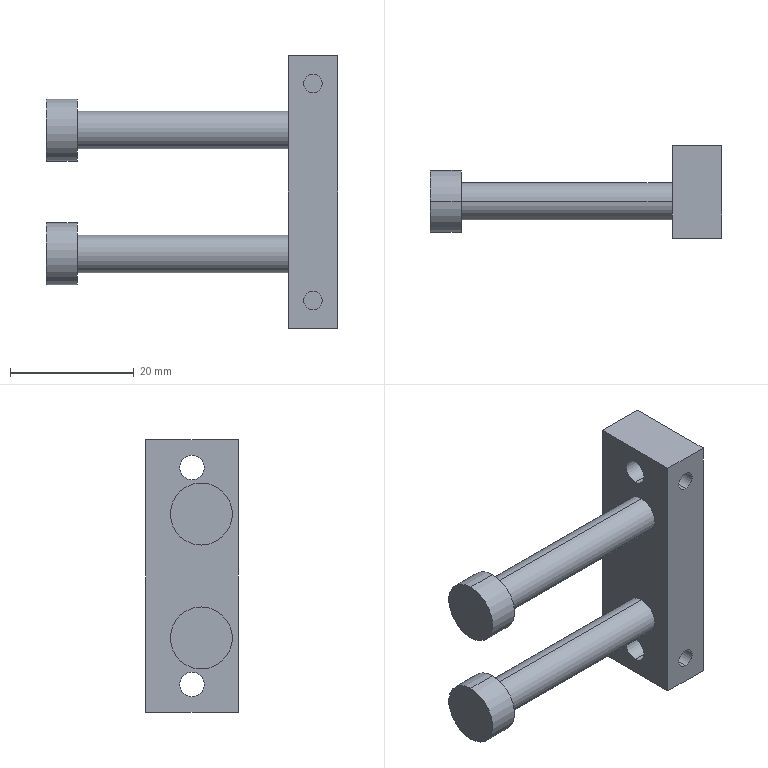Component | SolidWorks | F-YBExport-1-1_F-YBXCXSM10-15-Z73L-1_F-YBXCXSM10-15-Z73L_pr_cxs(PR_CXS_10-15)-1 | 1 solid | 34 faces | box 47 x 15 x 44 mm | volume 7646 mm3 | cylinder 20 | plane 14 | commonest cylinder face diameters 3 x8 10 x4 4 x4 6 x4
STEP:
#1=COLOUR_RGB('',0.7922,0.8196,0.9333);
#2=FILL_AREA_STYLE_COLOUR('',#1);
#3=FILL_AREA_STYLE('',(#2));
#4=SURFACE_STYLE_FILL_AREA(#3);
#5=SURFACE_SIDE_STYLE('',(#4));
#6=SURFACE_STYLE_USAGE(.BOTH.,#5);
#7=PRESENTATION_STYLE_ASSIGNMENT((#6));
#8=CARTESIAN_POINT('',(15.642,14.22,7.558));
#9=VERTEX_POINT('',#8);
#10=CARTESIAN_POINT('',(15.642,14.22,7.676));
#11=VERTEX_POINT('',#10);
#12=CARTESIAN_POINT('',(15.642,14.22,7.617));
#13=DIRECTION('',(0.,1.,0.));
#14=DIRECTION('',(0.,0.,-1.));
#15=AXIS2_PLACEMENT_3D('',#12,#13,#14);
#16=CIRCLE('',#15,0.05906);
#17=EDGE_CURVE('',#9,#11,#16,.T.);
#18=ORIENTED_EDGE('',*,*,#17,.T.);
#19=CARTESIAN_POINT('',(15.642,14.023,7.676));
#20=VERTEX_POINT('',#19);
#21=CARTESIAN_POINT('',(15.642,14.22,7.676));
#22=DIRECTION('',(0.,-1.,0.));
#23=VECTOR('',#22,39.37);
#24=LINE('',#21,#23);
#25=EDGE_CURVE('',#11,#20,#24,.T.);
#26=ORIENTED_EDGE('',*,*,#25,.T.);
#27=CARTESIAN_POINT('',(15.642,14.023,7.558));
#28=VERTEX_POINT('',#27);
#29=CARTESIAN_POINT('',(15.642,14.023,7.617));
#30=DIRECTION('',(0.,1.,0.));
#31=DIRECTION('',(0.,0.,-1.));
#32=AXIS2_PLACEMENT_3D('',#29,#30,#31);
#33=CIRCLE('',#32,0.05906);
#34=EDGE_CURVE('',#28,#20,#33,.T.);
#35=ORIENTED_EDGE('',*,*,#34,.F.);
#36=CARTESIAN_POINT('',(15.642,14.22,7.558));
#37=DIRECTION('',(0.,-1.,0.));
#38=VECTOR('',#37,39.37);
#39=LINE('',#36,#38);
#40=EDGE_CURVE('',#9,#28,#39,.T.);
#41=ORIENTED_EDGE('',*,*,#40,.F.);
#42=EDGE_LOOP('',(#18,#26,#35,#41));
#43=FACE_OUTER_BOUND('',#42,.T.);
#44=CARTESIAN_POINT('',(15.642,14.22,7.617));
#45=DIRECTION('',(0.,-1.,0.));
#46=DIRECTION('',(0.,0.,-1.));
#47=AXIS2_PLACEMENT_3D('',#44,#45,#46);
#48=CYLINDRICAL_SURFACE('',#47,0.05906);
#49=ADVANCED_FACE('',(#43),#48,.F.);
#50=CARTESIAN_POINT('',(15.642,14.22,6.18));
#51=VERTEX_POINT('',#50);
#52=CARTESIAN_POINT('',(15.642,14.22,6.298));
#53=VERTEX_POINT('',#52);
#54=CARTESIAN_POINT('',(15.642,14.22,6.239));
#55=DIRECTION('',(0.,1.,0.));
#56=DIRECTION('',(0.,0.,1.));
#57=AXIS2_PLACEMENT_3D('',#54,#55,#56);
#58=CIRCLE('',#57,0.05906);
#59=EDGE_CURVE('',#51,#53,#58,.T.);
#60=ORIENTED_EDGE('',*,*,#59,.T.);
#61=CARTESIAN_POINT('',(15.642,14.023,6.298));
#62=VERTEX_POINT('',#61);
#63=CARTESIAN_POINT('',(15.642,14.22,6.298));
#64=DIRECTION('',(0.,-1.,0.));
#65=VECTOR('',#64,39.37);
#66=LINE('',#63,#65);
#67=EDGE_CURVE('',#53,#62,#66,.T.);
#68=ORIENTED_EDGE('',*,*,#67,.T.);
#69=CARTESIAN_POINT('',(15.642,14.023,6.18));
#70=VERTEX_POINT('',#69);
#71=CARTESIAN_POINT('',(15.642,14.023,6.239));
#72=DIRECTION('',(0.,1.,0.));
#73=DIRECTION('',(0.,0.,1.));
#74=AXIS2_PLACEMENT_3D('',#71,#72,#73);
#75=CIRCLE('',#74,0.05906);
#76=EDGE_CURVE('',#70,#62,#75,.T.);
#77=ORIENTED_EDGE('',*,*,#76,.F.);
#78=CARTESIAN_POINT('',(15.642,14.22,6.18));
#79=DIRECTION('',(0.,-1.,0.));
#80=VECTOR('',#79,39.37);
#81=LINE('',#78,#80);
#82=EDGE_CURVE('',#51,#70,#81,.T.);
#83=ORIENTED_EDGE('',*,*,#82,.F.);
#84=EDGE_LOOP('',(#60,#68,#77,#83));
#85=FACE_OUTER_BOUND('',#84,.T.);
#86=CARTESIAN_POINT('',(15.642,14.22,6.239));
#87=DIRECTION('',(0.,-1.,0.));
#88=DIRECTION('',(0.,0.,-1.));
#89=AXIS2_PLACEMENT_3D('',#86,#87,#88);
#90=CYLINDRICAL_SURFACE('',#89,0.05906);
#91=ADVANCED_FACE('',(#85),#90,.F.);
#92=CARTESIAN_POINT('',(15.642,14.416,7.558));
#93=VERTEX_POINT('',#92);
#94=CARTESIAN_POINT('',(15.642,14.416,7.676));
#95=VERTEX_POINT('',#94);
#96=CARTESIAN_POINT('',(15.642,14.416,7.617));
#97=DIRECTION('',(0.,1.,0.));
#98=DIRECTION('',(0.,0.,-1.));
#99=AXIS2_PLACEMENT_3D('',#96,#97,#98);
#100=CIRCLE('',#99,0.05906);
#101=EDGE_CURVE('',#93,#95,#100,.T.);
#102=ORIENTED_EDGE('',*,*,#101,.F.);
#103=CARTESIAN_POINT('',(15.642,14.613,7.558));
#104=VERTEX_POINT('',#103);
#105=CARTESIAN_POINT('',(15.642,14.416,7.558));
#106=DIRECTION('',(0.,1.,0.));
#107=VECTOR('',#106,39.37);
#108=LINE('',#105,#107);
#109=EDGE_CURVE('',#93,#104,#108,.T.);
#110=ORIENTED_EDGE('',*,*,#109,.T.);
#111=CARTESIAN_POINT('',(15.642,14.613,7.676));
#112=VERTEX_POINT('',#111);
#113=CARTESIAN_POINT('',(15.642,14.613,7.617));
#114=DIRECTION('',(0.,1.,0.));
#115=DIRECTION('',(0.,0.,-1.));
#116=AXIS2_PLACEMENT_3D('',#113,#114,#115);
#117=CIRCLE('',#116,0.05906);
#118=EDGE_CURVE('',#104,#112,#117,.T.);
#119=ORIENTED_EDGE('',*,*,#118,.T.);
#120=CARTESIAN_POINT('',(15.642,14.416,7.676));
#121=DIRECTION('',(0.,1.,0.));
#122=VECTOR('',#121,39.37);
#123=LINE('',#120,#122);
#124=EDGE_CURVE('',#95,#112,#123,.T.);
#125=ORIENTED_EDGE('',*,*,#124,.F.);
#126=EDGE_LOOP('',(#102,#110,#119,#125));
#127=FACE_OUTER_BOUND('',#126,.T.);
#128=CARTESIAN_POINT('',(15.642,14.416,7.617));
#129=DIRECTION('',(0.,1.,0.));
#130=DIRECTION('',(0.,0.,1.));
#131=AXIS2_PLACEMENT_3D('',#128,#129,#130);
#132=CYLINDRICAL_SURFACE('',#131,0.05906);
#133=ADVANCED_FACE('',(#127),#132,.F.);
#134=CARTESIAN_POINT('',(15.642,14.416,6.18));
#135=VERTEX_POINT('',#134);
#136=CARTESIAN_POINT('',(15.642,14.416,6.298));
#137=VERTEX_POINT('',#136);
#138=CARTESIAN_POINT('',(15.642,14.416,6.239));
#139=DIRECTION('',(0.,1.,0.));
#140=DIRECTION('',(0.,0.,1.));
#141=AXIS2_PLACEMENT_3D('',#138,#139,#140);
#142=CIRCLE('',#141,0.05906);
#143=EDGE_CURVE('',#135,#137,#142,.T.);
#144=ORIENTED_EDGE('',*,*,#143,.F.);
#145=CARTESIAN_POINT('',(15.642,14.613,6.18));
#146=VERTEX_POINT('',#145);
#147=CARTESIAN_POINT('',(15.642,14.416,6.18));
#148=DIRECTION('',(0.,1.,0.));
#149=VECTOR('',#148,39.37);
#150=LINE('',#147,#149);
#151=EDGE_CURVE('',#135,#146,#150,.T.);
#152=ORIENTED_EDGE('',*,*,#151,.T.);
#153=CARTESIAN_POINT('',(15.642,14.613,6.298));
#154=VERTEX_POINT('',#153);
#155=CARTESIAN_POINT('',(15.642,14.613,6.239));
#156=DIRECTION('',(0.,1.,0.));
#157=DIRECTION('',(0.,0.,1.));
#158=AXIS2_PLACEMENT_3D('',#155,#156,#157);
#159=CIRCLE('',#158,0.05906);
#160=EDGE_CURVE('',#146,#154,#159,.T.);
#161=ORIENTED_EDGE('',*,*,#160,.T.);
#162=CARTESIAN_POINT('',(15.642,14.416,6.298));
#163=DIRECTION('',(0.,1.,0.));
#164=VECTOR('',#163,39.37);
#165=LINE('',#162,#164);
#166=EDGE_CURVE('',#137,#154,#165,.T.);
#167=ORIENTED_EDGE('',*,*,#166,.F.);
#168=EDGE_LOOP('',(#144,#152,#161,#167));
#169=FACE_OUTER_BOUND('',#168,.T.);
#170=CARTESIAN_POINT('',(15.642,14.416,6.239));
#171=DIRECTION('',(0.,1.,0.));
#172=DIRECTION('',(0.,0.,1.));
#173=AXIS2_PLACEMENT_3D('',#170,#171,#172);
#174=CYLINDRICAL_SURFACE('',#173,0.05906);
#175=ADVANCED_FACE('',(#169),#174,.F.);
#176=CARTESIAN_POINT('',(14.146,14.259,7.519));
#177=VERTEX_POINT('',#176);
#178=CARTESIAN_POINT('',(14.146,14.259,7.125));
#179=VERTEX_POINT('',#178);
#180=CARTESIAN_POINT('',(14.146,14.259,7.322));
#181=DIRECTION('',(-1.,0.,0.));
#182=DIRECTION('',(0.,0.,1.));
#183=AXIS2_PLACEMENT_3D('',#180,#181,#182);
#184=CIRCLE('',#183,0.1969);
#185=EDGE_CURVE('',#177,#179,#184,.T.);
#186=ORIENTED_EDGE('',*,*,#185,.T.);
#187=CARTESIAN_POINT('',(13.949,14.259,7.125));
#188=VERTEX_POINT('',#187);
#189=CARTESIAN_POINT('',(14.146,14.259,7.125));
#190=DIRECTION('',(-1.,0.,0.));
#191=VECTOR('',#190,39.37);
#192=LINE('',#189,#191);
#193=EDGE_CURVE('',#179,#188,#192,.T.);
#194=ORIENTED_EDGE('',*,*,#193,.T.);
#195=CARTESIAN_POINT('',(13.949,14.259,7.519));
#196=VERTEX_POINT('',#195);
#197=CARTESIAN_POINT('',(13.949,14.259,7.322));
#198=DIRECTION('',(-1.,0.,0.));
#199=DIRECTION('',(0.,0.,1.));
#200=AXIS2_PLACEMENT_3D('',#197,#198,#199);
#201=CIRCLE('',#200,0.1969);
#202=EDGE_CURVE('',#196,#188,#201,.T.);
#203=ORIENTED_EDGE('',*,*,#202,.F.);
#204=CARTESIAN_POINT('',(14.146,14.259,7.519));
#205=DIRECTION('',(-1.,0.,0.));
#206=VECTOR('',#205,39.37);
#207=LINE('',#204,#206);
#208=EDGE_CURVE('',#177,#196,#207,.T.);
#209=ORIENTED_EDGE('',*,*,#208,.F.);
#210=EDGE_LOOP('',(#186,#194,#203,#209));
#211=FACE_OUTER_BOUND('',#210,.T.);
#212=CARTESIAN_POINT('',(14.146,14.259,7.322));
#213=DIRECTION('',(-1.,0.,0.));
#214=DIRECTION('',(0.,0.,1.));
#215=AXIS2_PLACEMENT_3D('',#212,#213,#214);
#216=CYLINDRICAL_SURFACE('',#215,0.1969);
#217=ADVANCED_FACE('',(#211),#216,.T.);
#218=CARTESIAN_POINT('',(14.146,14.259,6.731));
#219=VERTEX_POINT('',#218);
#220=CARTESIAN_POINT('',(14.146,14.259,6.338));
#221=VERTEX_POINT('',#220);
#222=CARTESIAN_POINT('',(14.146,14.259,6.535));
#223=DIRECTION('',(-1.,0.,0.));
#224=DIRECTION('',(0.,0.,1.));
#225=AXIS2_PLACEMENT_3D('',#222,#223,#224);
#226=CIRCLE('',#225,0.1969);
#227=EDGE_CURVE('',#219,#221,#226,.T.);
#228=ORIENTED_EDGE('',*,*,#227,.T.);
#229=CARTESIAN_POINT('',(13.949,14.259,6.338));
#230=VERTEX_POINT('',#229);
#231=CARTESIAN_POINT('',(14.146,14.259,6.338));
#232=DIRECTION('',(-1.,0.,0.));
#233=VECTOR('',#232,39.37);
#234=LINE('',#231,#233);
#235=EDGE_CURVE('',#221,#230,#234,.T.);
#236=ORIENTED_EDGE('',*,*,#235,.T.);
#237=CARTESIAN_POINT('',(13.949,14.259,6.731));
#238=VERTEX_POINT('',#237);
#239=CARTESIAN_POINT('',(13.949,14.259,6.535));
#240=DIRECTION('',(-1.,0.,0.));
#241=DIRECTION('',(0.,0.,1.));
#242=AXIS2_PLACEMENT_3D('',#239,#240,#241);
#243=CIRCLE('',#242,0.1969);
#244=EDGE_CURVE('',#238,#230,#243,.T.);
#245=ORIENTED_EDGE('',*,*,#244,.F.);
#246=CARTESIAN_POINT('',(14.146,14.259,6.731));
#247=DIRECTION('',(-1.,0.,0.));
#248=VECTOR('',#247,39.37);
#249=LINE('',#246,#248);
#250=EDGE_CURVE('',#219,#238,#249,.T.);
#251=ORIENTED_EDGE('',*,*,#250,.F.);
#252=EDGE_LOOP('',(#228,#236,#245,#251));
#253=FACE_OUTER_BOUND('',#252,.T.);
#254=CARTESIAN_POINT('',(14.146,14.259,6.535));
#255=DIRECTION('',(-1.,0.,0.));
#256=DIRECTION('',(0.,0.,1.));
#257=AXIS2_PLACEMENT_3D('',#254,#255,#256);
#258=CYLINDRICAL_SURFACE('',#257,0.1969);
#259=ADVANCED_FACE('',(#253),#258,.T.);
#260=CARTESIAN_POINT('',(15.799,14.318,7.696));
#261=VERTEX_POINT('',#260);
#262=CARTESIAN_POINT('',(15.799,14.318,7.539));
#263=VERTEX_POINT('',#262);
#264=CARTESIAN_POINT('',(15.799,14.318,7.617));
#265=DIRECTION('',(1.,0.,0.));
#266=DIRECTION('',(0.,0.,-1.));
#267=AXIS2_PLACEMENT_3D('',#264,#265,#266);
#268=CIRCLE('',#267,0.07874);
#269=EDGE_CURVE('',#261,#263,#268,.T.);
#270=ORIENTED_EDGE('',*,*,#269,.T.);
#271=CARTESIAN_POINT('',(15.484,14.318,7.539));
#272=VERTEX_POINT('',#271);
#273=CARTESIAN_POINT('',(15.799,14.318,7.539));
#274=DIRECTION('',(-1.,0.,0.));
#275=VECTOR('',#274,39.37);
#276=LINE('',#273,#275);
#277=EDGE_CURVE('',#263,#272,#276,.T.);
#278=ORIENTED_EDGE('',*,*,#277,.T.);
#279=CARTESIAN_POINT('',(15.484,14.318,7.696));
#280=VERTEX_POINT('',#279);
#281=CARTESIAN_POINT('',(15.484,14.318,7.617));
#282=DIRECTION('',(1.,0.,0.));
#283=DIRECTION('',(0.,0.,-1.));
#284=AXIS2_PLACEMENT_3D('',#281,#282,#283);
#285=CIRCLE('',#284,0.07874);
#286=EDGE_CURVE('',#280,#272,#285,.T.);
#287=ORIENTED_EDGE('',*,*,#286,.F.);
#288=CARTESIAN_POINT('',(15.799,14.318,7.696));
#289=DIRECTION('',(-1.,0.,0.));
#290=VECTOR('',#289,39.37);
#291=LINE('',#288,#290);
#292=EDGE_CURVE('',#261,#280,#291,.T.);
#293=ORIENTED_EDGE('',*,*,#292,.F.);
#294=EDGE_LOOP('',(#270,#278,#287,#293));
#295=FACE_OUTER_BOUND('',#294,.T.);
#296=CARTESIAN_POINT('',(15.799,14.318,7.617));
#297=DIRECTION('',(-1.,0.,0.));
#298=DIRECTION('',(0.,0.,1.));
#299=AXIS2_PLACEMENT_3D('',#296,#297,#298);
#300=CYLINDRICAL_SURFACE('',#299,0.07874);
#301=ADVANCED_FACE('',(#295),#300,.F.);
#302=CARTESIAN_POINT('',(15.799,14.318,6.318));
#303=VERTEX_POINT('',#302);
#304=CARTESIAN_POINT('',(15.799,14.318,6.161));
#305=VERTEX_POINT('',#304);
#306=CARTESIAN_POINT('',(15.799,14.318,6.239));
#307=DIRECTION('',(1.,0.,0.));
#308=DIRECTION('',(0.,0.,-1.));
#309=AXIS2_PLACEMENT_3D('',#306,#307,#308);
#310=CIRCLE('',#309,0.07874);
#311=EDGE_CURVE('',#303,#305,#310,.T.);
#312=ORIENTED_EDGE('',*,*,#311,.T.);
#313=CARTESIAN_POINT('',(15.484,14.318,6.161));
#314=VERTEX_POINT('',#313);
#315=CARTESIAN_POINT('',(15.799,14.318,6.161));
#316=DIRECTION('',(-1.,0.,0.));
#317=VECTOR('',#316,39.37);
#318=LINE('',#315,#317);
#319=EDGE_CURVE('',#305,#314,#318,.T.);
#320=ORIENTED_EDGE('',*,*,#319,.T.);
#321=CARTESIAN_POINT('',(15.484,14.318,6.318));
#322=VERTEX_POINT('',#321);
#323=CARTESIAN_POINT('',(15.484,14.318,6.239));
#324=DIRECTION('',(1.,0.,0.));
#325=DIRECTION('',(0.,0.,-1.));
#326=AXIS2_PLACEMENT_3D('',#323,#324,#325);
#327=CIRCLE('',#326,0.07874);
#328=EDGE_CURVE('',#322,#314,#327,.T.);
#329=ORIENTED_EDGE('',*,*,#328,.F.);
#330=CARTESIAN_POINT('',(15.799,14.318,6.318));
#331=DIRECTION('',(-1.,0.,0.));
#332=VECTOR('',#331,39.37);
#333=LINE('',#330,#332);
#334=EDGE_CURVE('',#303,#322,#333,.T.);
#335=ORIENTED_EDGE('',*,*,#334,.F.);
#336=EDGE_LOOP('',(#312,#320,#329,#335));
#337=FACE_OUTER_BOUND('',#336,.T.);
#338=CARTESIAN_POINT('',(15.799,14.318,6.239));
#339=DIRECTION('',(-1.,0.,0.));
#340=DIRECTION('',(0.,0.,1.));
#341=AXIS2_PLACEMENT_3D('',#338,#339,#340);
#342=CYLINDRICAL_SURFACE('',#341,0.07874);
#343=ADVANCED_FACE('',(#337),#342,.F.);
#344=CARTESIAN_POINT('',(14.146,14.259,6.653));
#345=VERTEX_POINT('',#344);
#346=CARTESIAN_POINT('',(14.146,14.259,6.417));
#347=VERTEX_POINT('',#346);
#348=CARTESIAN_POINT('',(14.146,14.259,6.535));
#349=DIRECTION('',(-1.,0.,0.));
#350=DIRECTION('',(0.,0.,1.));
#351=AXIS2_PLACEMENT_3D('',#348,#349,#350);
#352=CIRCLE('',#351,0.1181);
#353=EDGE_CURVE('',#345,#347,#352,.T.);
#354=ORIENTED_EDGE('',*,*,#353,.F.);
#355=CARTESIAN_POINT('',(15.484,14.259,6.653));
#356=VERTEX_POINT('',#355);
#357=CARTESIAN_POINT('',(13.949,14.259,6.653));
#358=DIRECTION('',(1.,0.,0.));
#359=VECTOR('',#358,39.37);
#360=LINE('',#357,#359);
#361=EDGE_CURVE('',#345,#356,#360,.T.);
#362=ORIENTED_EDGE('',*,*,#361,.T.);
#363=CARTESIAN_POINT('',(15.484,14.259,6.417));
#364=VERTEX_POINT('',#363);
#365=CARTESIAN_POINT('',(15.484,14.259,6.535));
#366=DIRECTION('',(1.,0.,0.));
#367=DIRECTION('',(0.,0.,1.));
#368=AXIS2_PLACEMENT_3D('',#365,#366,#367);
#369=CIRCLE('',#368,0.1181);
#370=EDGE_CURVE('',#364,#356,#369,.T.);
#371=ORIENTED_EDGE('',*,*,#370,.F.);
#372=CARTESIAN_POINT('',(13.949,14.259,6.417));
#373=DIRECTION('',(1.,0.,0.));
#374=VECTOR('',#373,39.37);
#375=LINE('',#372,#374);
#376=EDGE_CURVE('',#347,#364,#375,.T.);
#377=ORIENTED_EDGE('',*,*,#376,.F.);
#378=EDGE_LOOP('',(#354,#362,#371,#377));
#379=FACE_OUTER_BOUND('',#378,.T.);
#380=CARTESIAN_POINT('',(13.949,14.259,6.535));
#381=DIRECTION('',(1.,0.,0.));
#382=DIRECTION('',(0.,0.,-1.));
#383=AXIS2_PLACEMENT_3D('',#380,#381,#382);
#384=CYLINDRICAL_SURFACE('',#383,0.1181);
#385=ADVANCED_FACE('',(#379),#384,.T.);
#386=CARTESIAN_POINT('',(14.146,14.259,7.44));
#387=VERTEX_POINT('',#386);
#388=CARTESIAN_POINT('',(14.146,14.259,7.204));
#389=VERTEX_POINT('',#388);
#390=CARTESIAN_POINT('',(14.146,14.259,7.322));
#391=DIRECTION('',(-1.,0.,0.));
#392=DIRECTION('',(0.,0.,1.));
#393=AXIS2_PLACEMENT_3D('',#390,#391,#392);
#394=CIRCLE('',#393,0.1181);
#395=EDGE_CURVE('',#387,#389,#394,.T.);
#396=ORIENTED_EDGE('',*,*,#395,.F.);
#397=CARTESIAN_POINT('',(15.484,14.259,7.44));
#398=VERTEX_POINT('',#397);
#399=CARTESIAN_POINT('',(13.949,14.259,7.44));
#400=DIRECTION('',(1.,0.,0.));
#401=VECTOR('',#400,39.37);
#402=LINE('',#399,#401);
#403=EDGE_CURVE('',#387,#398,#402,.T.);
#404=ORIENTED_EDGE('',*,*,#403,.T.);
#405=CARTESIAN_POINT('',(15.484,14.259,7.204));
#406=VERTEX_POINT('',#405);
#407=CARTESIAN_POINT('',(15.484,14.259,7.322));
#408=DIRECTION('',(1.,0.,0.));
#409=DIRECTION('',(0.,0.,1.));
#410=AXIS2_PLACEMENT_3D('',#407,#408,#409);
#411=CIRCLE('',#410,0.1181);
#412=EDGE_CURVE('',#406,#398,#411,.T.);
#413=ORIENTED_EDGE('',*,*,#412,.F.);
#414=CARTESIAN_POINT('',(13.949,14.259,7.204));
#415=DIRECTION('',(1.,0.,0.));
#416=VECTOR('',#415,39.37);
#417=LINE('',#414,#416);
#418=EDGE_CURVE('',#389,#406,#417,.T.);
#419=ORIENTED_EDGE('',*,*,#418,.F.);
#420=EDGE_LOOP('',(#396,#404,#413,#419));
#421=FACE_OUTER_BOUND('',#420,.T.);
#422=CARTESIAN_POINT('',(13.949,14.259,7.322));
#423=DIRECTION('',(1.,0.,0.));
#424=DIRECTION('',(0.,0.,-1.));
#425=AXIS2_PLACEMENT_3D('',#422,#423,#424);
#426=CYLINDRICAL_SURFACE('',#425,0.1181);
#427=ADVANCED_FACE('',(#421),#426,.T.);
#428=ORIENTED_EDGE('',*,*,#76,.T.);
#429=CARTESIAN_POINT('',(15.642,14.023,6.239));
#430=DIRECTION('',(0.,1.,0.));
#431=DIRECTION('',(0.,0.,1.));
#432=AXIS2_PLACEMENT_3D('',#429,#430,#431);
#433=CIRCLE('',#432,0.05906);
#434=EDGE_CURVE('',#62,#70,#433,.T.);
#435=ORIENTED_EDGE('',*,*,#434,.T.);
#436=EDGE_LOOP('',(#428,#435));
#437=FACE_BOUND('',#436,.T.);
#438=CARTESIAN_POINT('',(15.484,14.023,7.794));
#439=VERTEX_POINT('',#438);
#440=CARTESIAN_POINT('',(15.484,14.023,6.062));
#441=VERTEX_POINT('',#440);
#442=CARTESIAN_POINT('',(15.484,14.023,7.794));
#443=DIRECTION('',(0.,-0.,-1.));
#444=VECTOR('',#443,39.37);
#445=LINE('',#442,#444);
#446=EDGE_CURVE('',#439,#441,#445,.T.);
#447=ORIENTED_EDGE('',*,*,#446,.T.);
#448=CARTESIAN_POINT('',(15.799,14.023,6.062));
#449=VERTEX_POINT('',#448);
#450=CARTESIAN_POINT('',(15.799,14.023,6.062));
#451=DIRECTION('',(-1.,0.,0.));
#452=VECTOR('',#451,39.37);
#453=LINE('',#450,#452);
#454=EDGE_CURVE('',#449,#441,#453,.T.);
#455=ORIENTED_EDGE('',*,*,#454,.F.);
#456=CARTESIAN_POINT('',(15.799,14.023,7.794));
#457=VERTEX_POINT('',#456);
#458=CARTESIAN_POINT('',(15.799,14.023,7.794));
#459=DIRECTION('',(0.,-0.,-1.));
#460=VECTOR('',#459,39.37);
#461=LINE('',#458,#460);
#462=EDGE_CURVE('',#457,#449,#461,.T.);
#463=ORIENTED_EDGE('',*,*,#462,.F.);
#464=CARTESIAN_POINT('',(15.799,14.023,7.794));
#465=DIRECTION('',(-1.,0.,0.));
#466=VECTOR('',#465,39.37);
#467=LINE('',#464,#466);
#468=EDGE_CURVE('',#457,#439,#467,.T.);
#469=ORIENTED_EDGE('',*,*,#468,.T.);
#470=EDGE_LOOP('',(#447,#455,#463,#469));
#471=FACE_OUTER_BOUND('',#470,.T.);
#472=ORIENTED_EDGE('',*,*,#34,.T.);
#473=CARTESIAN_POINT('',(15.642,14.023,7.617));
#474=DIRECTION('',(0.,1.,0.));
#475=DIRECTION('',(0.,0.,-1.));
#476=AXIS2_PLACEMENT_3D('',#473,#474,#475);
#477=CIRCLE('',#476,0.05906);
#478=EDGE_CURVE('',#20,#28,#477,.T.);
#479=ORIENTED_EDGE('',*,*,#478,.T.);
#480=EDGE_LOOP('',(#472,#479));
#481=FACE_BOUND('',#480,.T.);
#482=CARTESIAN_POINT('',(15.799,14.023,7.794));
#483=DIRECTION('',(0.,1.,-0.));
#484=DIRECTION('',(0.,0.,1.));
#485=AXIS2_PLACEMENT_3D('',#482,#483,#484);
#486=PLANE('',#485);
#487=ADVANCED_FACE('',(#437,#471,#481),#486,.F.);
#488=ORIENTED_EDGE('',*,*,#403,.F.);
#489=CARTESIAN_POINT('',(14.146,14.259,7.322));
#490=DIRECTION('',(-1.,0.,0.));
#491=DIRECTION('',(0.,0.,1.));
#492=AXIS2_PLACEMENT_3D('',#489,#490,#491);
#493=CIRCLE('',#492,0.1181);
#494=EDGE_CURVE('',#389,#387,#493,.T.);
#495=ORIENTED_EDGE('',*,*,#494,.F.);
#496=ORIENTED_EDGE('',*,*,#418,.T.);
#497=CARTESIAN_POINT('',(15.484,14.259,7.322));
#498=DIRECTION('',(1.,0.,0.));
#499=DIRECTION('',(0.,0.,1.));
#500=AXIS2_PLACEMENT_3D('',#497,#498,#499);
#501=CIRCLE('',#500,0.1181);
#502=EDGE_CURVE('',#398,#406,#501,.T.);
#503=ORIENTED_EDGE('',*,*,#502,.F.);
#504=EDGE_LOOP('',(#488,#495,#496,#503));
#505=FACE_OUTER_BOUND('',#504,.T.);
#506=CARTESIAN_POINT('',(13.949,14.259,7.322));
#507=DIRECTION('',(1.,0.,0.));
#508=DIRECTION('',(0.,0.,-1.));
#509=AXIS2_PLACEMENT_3D('',#506,#507,#508);
#510=CYLINDRICAL_SURFACE('',#509,0.1181);
#511=ADVANCED_FACE('',(#505),#510,.T.);
#512=ORIENTED_EDGE('',*,*,#361,.F.);
#513=CARTESIAN_POINT('',(14.146,14.259,6.535));
#514=DIRECTION('',(-1.,0.,0.));
#515=DIRECTION('',(0.,0.,1.));
#516=AXIS2_PLACEMENT_3D('',#513,#514,#515);
#517=CIRCLE('',#516,0.1181);
#518=EDGE_CURVE('',#347,#345,#517,.T.);
#519=ORIENTED_EDGE('',*,*,#518,.F.);
#520=ORIENTED_EDGE('',*,*,#376,.T.);
#521=CARTESIAN_POINT('',(15.484,14.259,6.535));
#522=DIRECTION('',(1.,0.,0.));
#523=DIRECTION('',(0.,0.,1.));
#524=AXIS2_PLACEMENT_3D('',#521,#522,#523);
#525=CIRCLE('',#524,0.1181);
#526=EDGE_CURVE('',#356,#364,#525,.T.);
#527=ORIENTED_EDGE('',*,*,#526,.F.);
#528=EDGE_LOOP('',(#512,#519,#520,#527));
#529=FACE_OUTER_BOUND('',#528,.T.);
#530=CARTESIAN_POINT('',(13.949,14.259,6.535));
#531=DIRECTION('',(1.,0.,0.));
#532=DIRECTION('',(0.,0.,-1.));
#533=AXIS2_PLACEMENT_3D('',#530,#531,#532);
#534=CYLINDRICAL_SURFACE('',#533,0.1181);
#535=ADVANCED_FACE('',(#529),#534,.T.);
#536=ORIENTED_EDGE('',*,*,#370,.T.);
#537=ORIENTED_EDGE('',*,*,#526,.T.);
#538=EDGE_LOOP('',(#536,#537));
#539=FACE_BOUND('',#538,.T.);
#540=ORIENTED_EDGE('',*,*,#328,.T.);
#541=CARTESIAN_POINT('',(15.484,14.318,6.239));
#542=DIRECTION('',(1.,0.,0.));
#543=DIRECTION('',(0.,0.,-1.));
#544=AXIS2_PLACEMENT_3D('',#541,#542,#543);
#545=CIRCLE('',#544,0.07874);
#546=EDGE_CURVE('',#314,#322,#545,.T.);
#547=ORIENTED_EDGE('',*,*,#546,.T.);
#548=EDGE_LOOP('',(#540,#547));
#549=FACE_BOUND('',#548,.T.);
#550=CARTESIAN_POINT('',(15.484,14.613,6.062));
#551=VERTEX_POINT('',#550);
#552=CARTESIAN_POINT('',(15.484,14.613,7.794));
#553=VERTEX_POINT('',#552);
#554=CARTESIAN_POINT('',(15.484,14.613,6.062));
#555=DIRECTION('',(0.,-0.,1.));
#556=VECTOR('',#555,39.37);
#557=LINE('',#554,#556);
#558=EDGE_CURVE('',#551,#553,#557,.T.);
#559=ORIENTED_EDGE('',*,*,#558,.F.);
#560=CARTESIAN_POINT('',(15.484,14.023,6.062));
#561=DIRECTION('',(0.,1.,0.));
#562=VECTOR('',#561,39.37);
#563=LINE('',#560,#562);
#564=EDGE_CURVE('',#441,#551,#563,.T.);
#565=ORIENTED_EDGE('',*,*,#564,.F.);
#566=ORIENTED_EDGE('',*,*,#446,.F.);
#567=CARTESIAN_POINT('',(15.484,14.613,7.794));
#568=DIRECTION('',(0.,-1.,-0.));
#569=VECTOR('',#568,39.37);
#570=LINE('',#567,#569);
#571=EDGE_CURVE('',#553,#439,#570,.T.);
#572=ORIENTED_EDGE('',*,*,#571,.F.);
#573=EDGE_LOOP('',(#559,#565,#566,#572));
#574=FACE_OUTER_BOUND('',#573,.T.);
#575=ORIENTED_EDGE('',*,*,#286,.T.);
#576=CARTESIAN_POINT('',(15.484,14.318,7.617));
#577=DIRECTION('',(1.,0.,0.));
#578=DIRECTION('',(0.,0.,-1.));
#579=AXIS2_PLACEMENT_3D('',#576,#577,#578);
#580=CIRCLE('',#579,0.07874);
#581=EDGE_CURVE('',#272,#280,#580,.T.);
#582=ORIENTED_EDGE('',*,*,#581,.T.);
#583=EDGE_LOOP('',(#575,#582));
#584=FACE_BOUND('',#583,.T.);
#585=ORIENTED_EDGE('',*,*,#412,.T.);
#586=ORIENTED_EDGE('',*,*,#502,.T.);
#587=EDGE_LOOP('',(#585,#586));
#588=FACE_BOUND('',#587,.T.);
#589=CARTESIAN_POINT('',(15.484,14.613,6.062));
#590=DIRECTION('',(-1.,0.,0.));
#591=DIRECTION('',(0.,0.,1.));
#592=AXIS2_PLACEMENT_3D('',#589,#590,#591);
#593=PLANE('',#592);
#594=ADVANCED_FACE('',(#539,#549,#574,#584,#588),#593,.T.);
#595=ORIENTED_EDGE('',*,*,#311,.F.);
#596=CARTESIAN_POINT('',(15.799,14.318,6.239));
#597=DIRECTION('',(1.,0.,0.));
#598=DIRECTION('',(0.,0.,-1.));
#599=AXIS2_PLACEMENT_3D('',#596,#597,#598);
#600=CIRCLE('',#599,0.07874);
#601=EDGE_CURVE('',#305,#303,#600,.T.);
#602=ORIENTED_EDGE('',*,*,#601,.F.);
#603=EDGE_LOOP('',(#595,#602));
#604=FACE_BOUND('',#603,.T.);
#605=CARTESIAN_POINT('',(15.799,14.613,6.062));
#606=VERTEX_POINT('',#605);
#607=CARTESIAN_POINT('',(15.799,14.613,7.794));
#608=VERTEX_POINT('',#607);
#609=CARTESIAN_POINT('',(15.799,14.613,6.062));
#610=DIRECTION('',(0.,-0.,1.));
#611=VECTOR('',#610,39.37);
#612=LINE('',#609,#611);
#613=EDGE_CURVE('',#606,#608,#612,.T.);
#614=ORIENTED_EDGE('',*,*,#613,.T.);
#615=CARTESIAN_POINT('',(15.799,14.613,7.794));
#616=DIRECTION('',(0.,-1.,-0.));
#617=VECTOR('',#616,39.37);
#618=LINE('',#615,#617);
#619=EDGE_CURVE('',#608,#457,#618,.T.);
#620=ORIENTED_EDGE('',*,*,#619,.T.);
#621=ORIENTED_EDGE('',*,*,#462,.T.);
#622=CARTESIAN_POINT('',(15.799,14.023,6.062));
#623=DIRECTION('',(0.,1.,0.));
#624=VECTOR('',#623,39.37);
#625=LINE('',#622,#624);
#626=EDGE_CURVE('',#449,#606,#625,.T.);
#627=ORIENTED_EDGE('',*,*,#626,.T.);
#628=EDGE_LOOP('',(#614,#620,#621,#627));
#629=FACE_OUTER_BOUND('',#628,.T.);
#630=ORIENTED_EDGE('',*,*,#269,.F.);
#631=CARTESIAN_POINT('',(15.799,14.318,7.617));
#632=DIRECTION('',(1.,0.,0.));
#633=DIRECTION('',(0.,0.,-1.));
#634=AXIS2_PLACEMENT_3D('',#631,#632,#633);
#635=CIRCLE('',#634,0.07874);
#636=EDGE_CURVE('',#263,#261,#635,.T.);
#637=ORIENTED_EDGE('',*,*,#636,.F.);
#638=EDGE_LOOP('',(#630,#637));
#639=FACE_BOUND('',#638,.T.);
#640=CARTESIAN_POINT('',(15.799,14.613,6.062));
#641=DIRECTION('',(-1.,0.,0.));
#642=DIRECTION('',(0.,0.,1.));
#643=AXIS2_PLACEMENT_3D('',#640,#641,#642);
#644=PLANE('',#643);
#645=ADVANCED_FACE('',(#604,#629,#639),#644,.F.);
#646=CARTESIAN_POINT('',(15.642,14.613,7.617));
#647=DIRECTION('',(0.,1.,0.));
#648=DIRECTION('',(0.,0.,-1.));
#649=AXIS2_PLACEMENT_3D('',#646,#647,#648);
#650=CIRCLE('',#649,0.05906);
#651=EDGE_CURVE('',#112,#104,#650,.T.);
#652=ORIENTED_EDGE('',*,*,#651,.F.);
#653=ORIENTED_EDGE('',*,*,#118,.F.);
#654=EDGE_LOOP('',(#652,#653));
#655=FACE_BOUND('',#654,.T.);
#656=CARTESIAN_POINT('',(15.642,14.613,6.239));
#657=DIRECTION('',(0.,1.,0.));
#658=DIRECTION('',(0.,0.,1.));
#659=AXIS2_PLACEMENT_3D('',#656,#657,#658);
#660=CIRCLE('',#659,0.05906);
#661=EDGE_CURVE('',#154,#146,#660,.T.);
#662=ORIENTED_EDGE('',*,*,#661,.F.);
#663=ORIENTED_EDGE('',*,*,#160,.F.);
#664=EDGE_LOOP('',(#662,#663));
#665=FACE_BOUND('',#664,.T.);
#666=ORIENTED_EDGE('',*,*,#558,.T.);
#667=CARTESIAN_POINT('',(15.799,14.613,7.794));
#668=DIRECTION('',(-1.,0.,0.));
#669=VECTOR('',#668,39.37);
#670=LINE('',#667,#669);
#671=EDGE_CURVE('',#608,#553,#670,.T.);
#672=ORIENTED_EDGE('',*,*,#671,.F.);
#673=ORIENTED_EDGE('',*,*,#613,.F.);
#674=CARTESIAN_POINT('',(15.799,14.613,6.062));
#675=DIRECTION('',(-1.,0.,0.));
#676=VECTOR('',#675,39.37);
#677=LINE('',#674,#676);
#678=EDGE_CURVE('',#606,#551,#677,.T.);
#679=ORIENTED_EDGE('',*,*,#678,.T.);
#680=EDGE_LOOP('',(#666,#672,#673,#679));
#681=FACE_OUTER_BOUND('',#680,.T.);
#682=CARTESIAN_POINT('',(15.799,14.613,6.062));
#683=DIRECTION('',(0.,-1.,-0.));
#684=DIRECTION('',(0.,0.,-1.));
#685=AXIS2_PLACEMENT_3D('',#682,#683,#684);
#686=PLANE('',#685);
#687=ADVANCED_FACE('',(#655,#665,#681),#686,.F.);
#688=ORIENTED_EDGE('',*,*,#571,.T.);
#689=ORIENTED_EDGE('',*,*,#468,.F.);
#690=ORIENTED_EDGE('',*,*,#619,.F.);
#691=ORIENTED_EDGE('',*,*,#671,.T.);
#692=EDGE_LOOP('',(#688,#689,#690,#691));
#693=FACE_OUTER_BOUND('',#692,.T.);
#694=CARTESIAN_POINT('',(15.799,14.613,7.794));
#695=DIRECTION('',(0.,0.,-1.));
#696=DIRECTION('',(0.,1.,0.));
#697=AXIS2_PLACEMENT_3D('',#694,#695,#696);
#698=PLANE('',#697);
#699=ADVANCED_FACE('',(#693),#698,.F.);
#700=ORIENTED_EDGE('',*,*,#564,.T.);
#701=ORIENTED_EDGE('',*,*,#678,.F.);
#702=ORIENTED_EDGE('',*,*,#626,.F.);
#703=ORIENTED_EDGE('',*,*,#454,.T.);
#704=EDGE_LOOP('',(#700,#701,#702,#703));
#705=FACE_OUTER_BOUND('',#704,.T.);
#706=CARTESIAN_POINT('',(15.799,14.023,6.062));
#707=DIRECTION('',(0.,-0.,1.));
#708=DIRECTION('',(0.,-1.,-0.));
#709=AXIS2_PLACEMENT_3D('',#706,#707,#708);
#710=PLANE('',#709);
#711=ADVANCED_FACE('',(#705),#710,.F.);
#712=ORIENTED_EDGE('',*,*,#319,.F.);
#713=ORIENTED_EDGE('',*,*,#601,.T.);
#714=ORIENTED_EDGE('',*,*,#334,.T.);
#715=ORIENTED_EDGE('',*,*,#546,.F.);
#716=EDGE_LOOP('',(#712,#713,#714,#715));
#717=FACE_OUTER_BOUND('',#716,.T.);
#718=CARTESIAN_POINT('',(15.799,14.318,6.239));
#719=DIRECTION('',(-1.,0.,0.));
#720=DIRECTION('',(0.,0.,1.));
#721=AXIS2_PLACEMENT_3D('',#718,#719,#720);
#722=CYLINDRICAL_SURFACE('',#721,0.07874);
#723=ADVANCED_FACE('',(#717),#722,.F.);
#724=ORIENTED_EDGE('',*,*,#277,.F.);
#725=ORIENTED_EDGE('',*,*,#636,.T.);
#726=ORIENTED_EDGE('',*,*,#292,.T.);
#727=ORIENTED_EDGE('',*,*,#581,.F.);
#728=EDGE_LOOP('',(#724,#725,#726,#727));
#729=FACE_OUTER_BOUND('',#728,.T.);
#730=CARTESIAN_POINT('',(15.799,14.318,7.617));
#731=DIRECTION('',(-1.,0.,0.));
#732=DIRECTION('',(0.,0.,1.));
#733=AXIS2_PLACEMENT_3D('',#730,#731,#732);
#734=CYLINDRICAL_SURFACE('',#733,0.07874);
#735=ADVANCED_FACE('',(#729),#734,.F.);
#736=ORIENTED_EDGE('',*,*,#227,.F.);
#737=CARTESIAN_POINT('',(14.146,14.259,6.535));
#738=DIRECTION('',(-1.,0.,0.));
#739=DIRECTION('',(0.,0.,1.));
#740=AXIS2_PLACEMENT_3D('',#737,#738,#739);
#741=CIRCLE('',#740,0.1969);
#742=EDGE_CURVE('',#221,#219,#741,.T.);
#743=ORIENTED_EDGE('',*,*,#742,.F.);
#744=EDGE_LOOP('',(#736,#743));
#745=FACE_OUTER_BOUND('',#744,.T.);
#746=ORIENTED_EDGE('',*,*,#518,.T.);
#747=ORIENTED_EDGE('',*,*,#353,.T.);
#748=EDGE_LOOP('',(#746,#747));
#749=FACE_BOUND('',#748,.T.);
#750=CARTESIAN_POINT('',(14.146,14.259,6.535));
#751=DIRECTION('',(-1.,0.,0.));
#752=DIRECTION('',(0.,0.,1.));
#753=AXIS2_PLACEMENT_3D('',#750,#751,#752);
#754=PLANE('',#753);
#755=ADVANCED_FACE('',(#745,#749),#754,.F.);
#756=ORIENTED_EDGE('',*,*,#235,.F.);
#757=ORIENTED_EDGE('',*,*,#742,.T.);
#758=ORIENTED_EDGE('',*,*,#250,.T.);
#759=CARTESIAN_POINT('',(13.949,14.259,6.535));
#760=DIRECTION('',(-1.,0.,0.));
#761=DIRECTION('',(0.,0.,1.));
#762=AXIS2_PLACEMENT_3D('',#759,#760,#761);
#763=CIRCLE('',#762,0.1969);
#764=EDGE_CURVE('',#230,#238,#763,.T.);
#765=ORIENTED_EDGE('',*,*,#764,.F.);
#766=EDGE_LOOP('',(#756,#757,#758,#765));
#767=FACE_OUTER_BOUND('',#766,.T.);
#768=CARTESIAN_POINT('',(14.146,14.259,6.535));
#769=DIRECTION('',(-1.,0.,0.));
#770=DIRECTION('',(0.,0.,1.));
#771=AXIS2_PLACEMENT_3D('',#768,#769,#770);
#772=CYLINDRICAL_SURFACE('',#771,0.1969);
#773=ADVANCED_FACE('',(#767),#772,.T.);
#774=ORIENTED_EDGE('',*,*,#244,.T.);
#775=ORIENTED_EDGE('',*,*,#764,.T.);
#776=EDGE_LOOP('',(#774,#775));
#777=FACE_OUTER_BOUND('',#776,.T.);
#778=CARTESIAN_POINT('',(13.949,14.259,6.535));
#779=DIRECTION('',(-1.,0.,0.));
#780=DIRECTION('',(0.,0.,1.));
#781=AXIS2_PLACEMENT_3D('',#778,#779,#780);
#782=PLANE('',#781);
#783=ADVANCED_FACE('',(#777),#782,.T.);
#784=ORIENTED_EDGE('',*,*,#185,.F.);
#785=CARTESIAN_POINT('',(14.146,14.259,7.322));
#786=DIRECTION('',(-1.,0.,0.));
#787=DIRECTION('',(0.,0.,1.));
#788=AXIS2_PLACEMENT_3D('',#785,#786,#787);
#789=CIRCLE('',#788,0.1969);
#790=EDGE_CURVE('',#179,#177,#789,.T.);
#791=ORIENTED_EDGE('',*,*,#790,.F.);
#792=EDGE_LOOP('',(#784,#791));
#793=FACE_OUTER_BOUND('',#792,.T.);
#794=ORIENTED_EDGE('',*,*,#494,.T.);
#795=ORIENTED_EDGE('',*,*,#395,.T.);
#796=EDGE_LOOP('',(#794,#795));
#797=FACE_BOUND('',#796,.T.);
#798=CARTESIAN_POINT('',(14.146,14.259,7.322));
#799=DIRECTION('',(-1.,0.,0.));
#800=DIRECTION('',(0.,0.,1.));
#801=AXIS2_PLACEMENT_3D('',#798,#799,#800);
#802=PLANE('',#801);
#803=ADVANCED_FACE('',(#793,#797),#802,.F.);
#804=ORIENTED_EDGE('',*,*,#193,.F.);
#805=ORIENTED_EDGE('',*,*,#790,.T.);
#806=ORIENTED_EDGE('',*,*,#208,.T.);
#807=CARTESIAN_POINT('',(13.949,14.259,7.322));
#808=DIRECTION('',(-1.,0.,0.));
#809=DIRECTION('',(0.,0.,1.));
#810=AXIS2_PLACEMENT_3D('',#807,#808,#809);
#811=CIRCLE('',#810,0.1969);
#812=EDGE_CURVE('',#188,#196,#811,.T.);
#813=ORIENTED_EDGE('',*,*,#812,.F.);
#814=EDGE_LOOP('',(#804,#805,#806,#813));
#815=FACE_OUTER_BOUND('',#814,.T.);
#816=CARTESIAN_POINT('',(14.146,14.259,7.322));
#817=DIRECTION('',(-1.,0.,0.));
#818=DIRECTION('',(0.,0.,1.));
#819=AXIS2_PLACEMENT_3D('',#816,#817,#818);
#820=CYLINDRICAL_SURFACE('',#819,0.1969);
#821=ADVANCED_FACE('',(#815),#820,.T.);
#822=ORIENTED_EDGE('',*,*,#202,.T.);
#823=ORIENTED_EDGE('',*,*,#812,.T.);
#824=EDGE_LOOP('',(#822,#823));
#825=FACE_OUTER_BOUND('',#824,.T.);
#826=CARTESIAN_POINT('',(13.949,14.259,7.322));
#827=DIRECTION('',(1.,0.,0.));
#828=DIRECTION('',(0.,0.,-1.));
#829=AXIS2_PLACEMENT_3D('',#826,#827,#828);
#830=PLANE('',#829);
#831=ADVANCED_FACE('',(#825),#830,.F.);
#832=ORIENTED_EDGE('',*,*,#151,.F.);
#833=CARTESIAN_POINT('',(15.642,14.416,6.239));
#834=DIRECTION('',(0.,1.,0.));
#835=DIRECTION('',(0.,0.,1.));
#836=AXIS2_PLACEMENT_3D('',#833,#834,#835);
#837=CIRCLE('',#836,0.05906);
#838=EDGE_CURVE('',#137,#135,#837,.T.);
#839=ORIENTED_EDGE('',*,*,#838,.F.);
#840=ORIENTED_EDGE('',*,*,#166,.T.);
#841=ORIENTED_EDGE('',*,*,#661,.T.);
#842=EDGE_LOOP('',(#832,#839,#840,#841));
#843=FACE_OUTER_BOUND('',#842,.T.);
#844=CARTESIAN_POINT('',(15.642,14.416,6.239));
#845=DIRECTION('',(0.,1.,0.));
#846=DIRECTION('',(0.,0.,1.));
#847=AXIS2_PLACEMENT_3D('',#844,#845,#846);
#848=CYLINDRICAL_SURFACE('',#847,0.05906);
#849=ADVANCED_FACE('',(#843),#848,.F.);
#850=ORIENTED_EDGE('',*,*,#838,.T.);
#851=ORIENTED_EDGE('',*,*,#143,.T.);
#852=EDGE_LOOP('',(#850,#851));
#853=FACE_OUTER_BOUND('',#852,.T.);
#854=CARTESIAN_POINT('',(15.642,14.416,6.239));
#855=DIRECTION('',(0.,1.,0.));
#856=DIRECTION('',(0.,0.,1.));
#857=AXIS2_PLACEMENT_3D('',#854,#855,#856);
#858=PLANE('',#857);
#859=ADVANCED_FACE('',(#853),#858,.T.);
#860=ORIENTED_EDGE('',*,*,#109,.F.);
#861=CARTESIAN_POINT('',(15.642,14.416,7.617));
#862=DIRECTION('',(0.,1.,0.));
#863=DIRECTION('',(0.,0.,-1.));
#864=AXIS2_PLACEMENT_3D('',#861,#862,#863);
#865=CIRCLE('',#864,0.05906);
#866=EDGE_CURVE('',#95,#93,#865,.T.);
#867=ORIENTED_EDGE('',*,*,#866,.F.);
#868=ORIENTED_EDGE('',*,*,#124,.T.);
#869=ORIENTED_EDGE('',*,*,#651,.T.);
#870=EDGE_LOOP('',(#860,#867,#868,#869));
#871=FACE_OUTER_BOUND('',#870,.T.);
#872=CARTESIAN_POINT('',(15.642,14.416,7.617));
#873=DIRECTION('',(0.,1.,0.));
#874=DIRECTION('',(0.,0.,1.));
#875=AXIS2_PLACEMENT_3D('',#872,#873,#874);
#876=CYLINDRICAL_SURFACE('',#875,0.05906);
#877=ADVANCED_FACE('',(#871),#876,.F.);
#878=ORIENTED_EDGE('',*,*,#866,.T.);
#879=ORIENTED_EDGE('',*,*,#101,.T.);
#880=EDGE_LOOP('',(#878,#879));
#881=FACE_OUTER_BOUND('',#880,.T.);
#882=CARTESIAN_POINT('',(15.642,14.416,7.617));
#883=DIRECTION('',(0.,-1.,0.));
#884=DIRECTION('',(0.,0.,-1.));
#885=AXIS2_PLACEMENT_3D('',#882,#883,#884);
#886=PLANE('',#885);
#887=ADVANCED_FACE('',(#881),#886,.F.);
#888=ORIENTED_EDGE('',*,*,#67,.F.);
#889=CARTESIAN_POINT('',(15.642,14.22,6.239));
#890=DIRECTION('',(0.,1.,0.));
#891=DIRECTION('',(0.,0.,1.));
#892=AXIS2_PLACEMENT_3D('',#889,#890,#891);
#893=CIRCLE('',#892,0.05906);
#894=EDGE_CURVE('',#53,#51,#893,.T.);
#895=ORIENTED_EDGE('',*,*,#894,.T.);
#896=ORIENTED_EDGE('',*,*,#82,.T.);
#897=ORIENTED_EDGE('',*,*,#434,.F.);
#898=EDGE_LOOP('',(#888,#895,#896,#897));
#899=FACE_OUTER_BOUND('',#898,.T.);
#900=CARTESIAN_POINT('',(15.642,14.22,6.239));
#901=DIRECTION('',(0.,-1.,0.));
#902=DIRECTION('',(0.,0.,-1.));
#903=AXIS2_PLACEMENT_3D('',#900,#901,#902);
#904=CYLINDRICAL_SURFACE('',#903,0.05906);
#905=ADVANCED_FACE('',(#899),#904,.F.);
#906=ORIENTED_EDGE('',*,*,#59,.F.);
#907=ORIENTED_EDGE('',*,*,#894,.F.);
#908=EDGE_LOOP('',(#906,#907));
#909=FACE_OUTER_BOUND('',#908,.T.);
#910=CARTESIAN_POINT('',(15.642,14.22,6.239));
#911=DIRECTION('',(0.,-1.,0.));
#912=DIRECTION('',(0.,0.,1.));
#913=AXIS2_PLACEMENT_3D('',#910,#911,#912);
#914=PLANE('',#913);
#915=ADVANCED_FACE('',(#909),#914,.T.);
#916=ORIENTED_EDGE('',*,*,#25,.F.);
#917=CARTESIAN_POINT('',(15.642,14.22,7.617));
#918=DIRECTION('',(0.,1.,0.));
#919=DIRECTION('',(0.,0.,-1.));
#920=AXIS2_PLACEMENT_3D('',#917,#918,#919);
#921=CIRCLE('',#920,0.05906);
#922=EDGE_CURVE('',#11,#9,#921,.T.);
#923=ORIENTED_EDGE('',*,*,#922,.T.);
#924=ORIENTED_EDGE('',*,*,#40,.T.);
#925=ORIENTED_EDGE('',*,*,#478,.F.);
#926=EDGE_LOOP('',(#916,#923,#924,#925));
#927=FACE_OUTER_BOUND('',#926,.T.);
#928=CARTESIAN_POINT('',(15.642,14.22,7.617));
#929=DIRECTION('',(0.,-1.,0.));
#930=DIRECTION('',(0.,0.,-1.));
#931=AXIS2_PLACEMENT_3D('',#928,#929,#930);
#932=CYLINDRICAL_SURFACE('',#931,0.05906);
#933=ADVANCED_FACE('',(#927),#932,.F.);
#934=ORIENTED_EDGE('',*,*,#17,.F.);
#935=ORIENTED_EDGE('',*,*,#922,.F.);
#936=EDGE_LOOP('',(#934,#935));
#937=FACE_OUTER_BOUND('',#936,.T.);
#938=CARTESIAN_POINT('',(15.642,14.22,7.617));
#939=DIRECTION('',(0.,1.,0.));
#940=DIRECTION('',(0.,0.,-1.));
#941=AXIS2_PLACEMENT_3D('',#938,#939,#940);
#942=PLANE('',#941);
#943=ADVANCED_FACE('',(#937),#942,.F.);
#944=CLOSED_SHELL('',(#49,#91,#133,#175,#217,#259,#301,#343,#385,#427,#487,#511,#535,#594,#645,#687,#699,#711,#723,#735,#755,#773,#783,#803,#821,#831,#849,#859,#877,#887,#905,#915,#933,#943));
#945=MANIFOLD_SOLID_BREP('',#944);
#946=STYLED_ITEM('',(#7),#945);
#947=PRESENTATION_LAYER_ASSIGNMENT('','',(#946));
#948=(LENGTH_UNIT()NAMED_UNIT(*)SI_UNIT($,.METRE.));
#949=LENGTH_MEASURE_WITH_UNIT(LENGTH_MEASURE(0.0254),#948);
#950=DIMENSIONAL_EXPONENTS(1.,0.,0.,0.,0.,0.,0.);
#951=(CONVERSION_BASED_UNIT('',#949)LENGTH_UNIT()NAMED_UNIT(#950));
#952=UNCERTAINTY_MEASURE_WITH_UNIT(LENGTH_MEASURE(0.00001),#951,'','');
#953=(NAMED_UNIT(*)PLANE_ANGLE_UNIT()SI_UNIT($,.RADIAN.));
#954=(NAMED_UNIT(*)SI_UNIT($,.STERADIAN.)SOLID_ANGLE_UNIT());
#955=(GEOMETRIC_REPRESENTATION_CONTEXT(3)GLOBAL_UNCERTAINTY_ASSIGNED_CONTEXT((#952))GLOBAL_UNIT_ASSIGNED_CONTEXT((#951,#953,#954))REPRESENTATION_CONTEXT('',''));
#956=MECHANICAL_DESIGN_GEOMETRIC_PRESENTATION_REPRESENTATION('',(#946),#955);
#957=CARTESIAN_POINT('',(0.,0.,0.));
#958=DIRECTION('',(0.,0.,1.));
#959=DIRECTION('',(1.,0.,0.));
#960=AXIS2_PLACEMENT_3D('',#957,#958,#959);
#961=(LENGTH_UNIT()NAMED_UNIT(*)SI_UNIT($,.METRE.));
#962=LENGTH_MEASURE_WITH_UNIT(LENGTH_MEASURE(0.0254),#961);
#963=DIMENSIONAL_EXPONENTS(1.,0.,0.,0.,0.,0.,0.);
#964=(CONVERSION_BASED_UNIT('',#962)LENGTH_UNIT()NAMED_UNIT(#963));
#965=UNCERTAINTY_MEASURE_WITH_UNIT(LENGTH_MEASURE(0.00001),#964,'','');
#966=(NAMED_UNIT(*)PLANE_ANGLE_UNIT()SI_UNIT($,.RADIAN.));
#967=(NAMED_UNIT(*)SI_UNIT($,.STERADIAN.)SOLID_ANGLE_UNIT());
#968=(GEOMETRIC_REPRESENTATION_CONTEXT(3)GLOBAL_UNCERTAINTY_ASSIGNED_CONTEXT((#965))GLOBAL_UNIT_ASSIGNED_CONTEXT((#964,#966,#967))REPRESENTATION_CONTEXT('',''));
#969=ADVANCED_BREP_SHAPE_REPRESENTATION('',(#945,#960),#968);